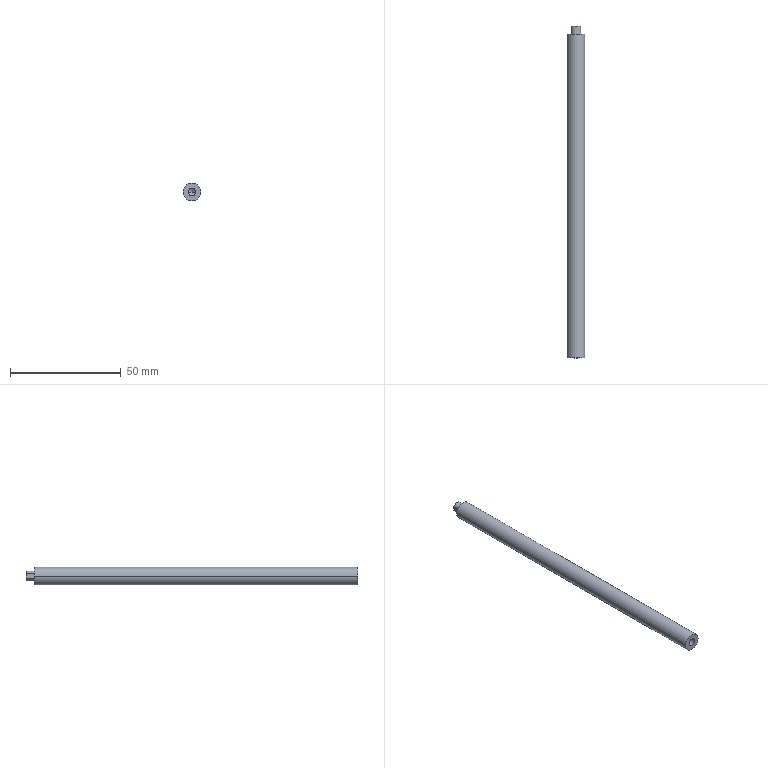Component | SolidWorks | 04LowerMaterialReceivingSwingAngleAssembly(3920)-1_04LowerMaterialReceivingDieAssembly(3920)-1_H2020022-0402-1-1 | 1 solid | 16 faces | box 8 x 150 x 8 mm | volume 7256 mm3 | cylinder 8 | cone 4 | plane 4 | commonest cylinder face diameters 3.3 x2 2.5 x2 4.5 x2 8 x2 | material 45#Steel
build123d program:
from build123d import *

# Parameters (mm, degrees)
SKETCH1_R             = 4
BOSS_EXTRUDE1_DEPTH   = 150
SKETCH2_OUTSIDE_W     = 40.086
SKETCH2_OUTSIDE_H     = 40.086
SKETCH2_OUTSIDE_R     = 2.25
CUT_EXTRUDE1_DEPTH    = 3.8
SKETCH3_W             = 6
SKETCH3_H             = 2
CUT_EXTRUDE2_DEPTH    = 3.8
M3_TAPPED_HOLE1_D     = 2.5
M3_TAPPED_HOLE1_DEPTH = 7.5
M3_TAPPED_HOLE1_TIP   = 0.7511
M4_TAPPED_HOLE1_D     = 3.3
M4_TAPPED_HOLE1_DEPTH = 13
M4_TAPPED_HOLE1_TIP   = 0.9914


with BuildPart() as part:
    # Sketch1 → Boss-Extrude1 (new body)
    with BuildSketch(Plane(origin=(0, 0, 0), x_dir=(1, 0, 0), z_dir=(0, 1, 0))):
        with Locations(Location((0, 0, 0), (0, 0, 270))):
            Circle(SKETCH1_R)
    extrude(amount=BOSS_EXTRUDE1_DEPTH)

    # Sketch2 outside → Cut-Extrude1 (cut)
    with BuildSketch(Plane(origin=(0, 150, 0), x_dir=(1, 0, 0), z_dir=(0, 1, 0))):
        Rectangle(SKETCH2_OUTSIDE_W, SKETCH2_OUTSIDE_H)
        with Locations(Location((0, 0, 0), (0, 0, 270))):
            Circle(SKETCH2_OUTSIDE_R, mode=Mode.SUBTRACT)
    extrude(amount=-CUT_EXTRUDE1_DEPTH, mode=Mode.SUBTRACT)

    # Sketch3 → Cut-Extrude2 (cut)
    with BuildSketch(Plane(origin=(0, 150, 0), x_dir=(1, 0, 0), z_dir=(0, 1, 0))):
        with Locations((0, 3)):
            Rectangle(SKETCH3_W, SKETCH3_H)
    extrude(amount=-CUT_EXTRUDE2_DEPTH, mode=Mode.SUBTRACT)

    # M3 Tapped Hole1
    with Locations(Plane(origin=(0, 150, 0), x_dir=(1, 0, 0), z_dir=(0, 1, 0))):
        with Locations((0, 0)):
            Hole(M3_TAPPED_HOLE1_D / 2, depth=M3_TAPPED_HOLE1_DEPTH)
            with Locations((0, 0, -(M3_TAPPED_HOLE1_DEPTH + M3_TAPPED_HOLE1_TIP / 2))):  # 118° drill point
                Cone(0, M3_TAPPED_HOLE1_D / 2, M3_TAPPED_HOLE1_TIP, mode=Mode.SUBTRACT)

    # M4 Tapped Hole1
    with Locations(Plane(origin=(0, 0, 0), x_dir=(-1, 0, 0), z_dir=(0, -1, 0))):
        with Locations((0, 0)):
            Hole(M4_TAPPED_HOLE1_D / 2, depth=M4_TAPPED_HOLE1_DEPTH)
            with Locations((0, 0, -(M4_TAPPED_HOLE1_DEPTH + M4_TAPPED_HOLE1_TIP / 2))):  # 118° drill point
                Cone(0, M4_TAPPED_HOLE1_D / 2, M4_TAPPED_HOLE1_TIP, mode=Mode.SUBTRACT)


solid = part.part

# Placed as in the assembly
solid = solid.moved(Location((0.03579, 124.813, 280.197), (0, 90, 0)))
STEP:
#1=COLOUR_RGB('',0.7922,0.8196,0.9333);
#2=FILL_AREA_STYLE_COLOUR('',#1);
#3=FILL_AREA_STYLE('',(#2));
#4=SURFACE_STYLE_FILL_AREA(#3);
#5=SURFACE_SIDE_STYLE('',(#4));
#6=SURFACE_STYLE_USAGE(.BOTH.,#5);
#7=PRESENTATION_STYLE_ASSIGNMENT((#6));
#8=CARTESIAN_POINT('',(0.06637,5.426,11.031));
#9=VERTEX_POINT('',#8);
#10=CARTESIAN_POINT('',(-0.06355,5.426,11.031));
#11=VERTEX_POINT('',#10);
#12=CARTESIAN_POINT('',(0.001409,5.426,11.031));
#13=DIRECTION('',(0.,-1.,0.));
#14=DIRECTION('',(-1.,0.,0.));
#15=AXIS2_PLACEMENT_3D('',#12,#13,#14);
#16=CIRCLE('',#15,0.06496);
#17=EDGE_CURVE('',#9,#11,#16,.T.);
#18=ORIENTED_EDGE('',*,*,#17,.F.);
#19=CARTESIAN_POINT('',(0.06637,4.914,11.031));
#20=VERTEX_POINT('',#19);
#21=CARTESIAN_POINT('',(0.06637,4.914,11.031));
#22=DIRECTION('',(0.,-1.,0.));
#23=VECTOR('',#22,39.37);
#24=LINE('',#21,#23);
#25=EDGE_CURVE('',#9,#20,#24,.T.);
#26=ORIENTED_EDGE('',*,*,#25,.T.);
#27=CARTESIAN_POINT('',(-0.06355,4.914,11.031));
#28=VERTEX_POINT('',#27);
#29=CARTESIAN_POINT('',(0.001409,4.914,11.031));
#30=DIRECTION('',(0.,-1.,0.));
#31=DIRECTION('',(-1.,0.,0.));
#32=AXIS2_PLACEMENT_3D('',#29,#30,#31);
#33=CIRCLE('',#32,0.06496);
#34=EDGE_CURVE('',#20,#28,#33,.T.);
#35=ORIENTED_EDGE('',*,*,#34,.T.);
#36=CARTESIAN_POINT('',(-0.06355,4.914,11.031));
#37=DIRECTION('',(0.,-1.,0.));
#38=VECTOR('',#37,39.37);
#39=LINE('',#36,#38);
#40=EDGE_CURVE('',#11,#28,#39,.T.);
#41=ORIENTED_EDGE('',*,*,#40,.F.);
#42=EDGE_LOOP('',(#18,#26,#35,#41));
#43=FACE_OUTER_BOUND('',#42,.T.);
#44=CARTESIAN_POINT('',(0.001409,4.914,11.031));
#45=DIRECTION('',(0.,-1.,0.));
#46=DIRECTION('',(-1.,0.,0.));
#47=AXIS2_PLACEMENT_3D('',#44,#45,#46);
#48=CYLINDRICAL_SURFACE('',#47,0.06496);
#49=ADVANCED_FACE('',(#43),#48,.F.);
#50=CARTESIAN_POINT('',(0.001409,5.465,11.031));
#51=VERTEX_POINT('',#50);
#52=CARTESIAN_POINT('',(-0.06355,5.426,11.031));
#53=DIRECTION('',(-0.8572,-0.515,0.));
#54=VECTOR('',#53,39.37);
#55=LINE('',#52,#54);
#56=EDGE_CURVE('',#51,#11,#55,.T.);
#57=ORIENTED_EDGE('',*,*,#56,.F.);
#58=CARTESIAN_POINT('',(0.06637,5.426,11.031));
#59=DIRECTION('',(0.8572,-0.515,-0.));
#60=VECTOR('',#59,39.37);
#61=LINE('',#58,#60);
#62=EDGE_CURVE('',#51,#9,#61,.T.);
#63=ORIENTED_EDGE('',*,*,#62,.T.);
#64=ORIENTED_EDGE('',*,*,#17,.T.);
#65=EDGE_LOOP('',(#57,#63,#64));
#66=FACE_OUTER_BOUND('',#65,.T.);
#67=CARTESIAN_POINT('',(0.001409,5.426,11.031));
#68=DIRECTION('',(0.,-1.,0.));
#69=DIRECTION('',(-1.,0.,0.));
#70=AXIS2_PLACEMENT_3D('',#67,#68,#69);
#71=CONICAL_SURFACE('',#70,0.06496,1.03);
#72=ADVANCED_FACE('',(#66),#71,.F.);
#73=CARTESIAN_POINT('',(-0.0478,10.524,11.031));
#74=VERTEX_POINT('',#73);
#75=CARTESIAN_POINT('',(0.05062,10.524,11.031));
#76=VERTEX_POINT('',#75);
#77=CARTESIAN_POINT('',(0.001409,10.524,11.031));
#78=DIRECTION('',(0.,1.,0.));
#79=DIRECTION('',(1.,0.,0.));
#80=AXIS2_PLACEMENT_3D('',#77,#78,#79);
#81=CIRCLE('',#80,0.04921);
#82=EDGE_CURVE('',#74,#76,#81,.T.);
#83=ORIENTED_EDGE('',*,*,#82,.F.);
#84=CARTESIAN_POINT('',(-0.0478,10.819,11.031));
#85=VERTEX_POINT('',#84);
#86=CARTESIAN_POINT('',(-0.0478,10.819,11.031));
#87=DIRECTION('',(0.,1.,0.));
#88=VECTOR('',#87,39.37);
#89=LINE('',#86,#88);
#90=EDGE_CURVE('',#74,#85,#89,.T.);
#91=ORIENTED_EDGE('',*,*,#90,.T.);
#92=CARTESIAN_POINT('',(0.05062,10.819,11.031));
#93=VERTEX_POINT('',#92);
#94=CARTESIAN_POINT('',(0.001409,10.819,11.031));
#95=DIRECTION('',(0.,1.,0.));
#96=DIRECTION('',(1.,0.,0.));
#97=AXIS2_PLACEMENT_3D('',#94,#95,#96);
#98=CIRCLE('',#97,0.04921);
#99=EDGE_CURVE('',#85,#93,#98,.T.);
#100=ORIENTED_EDGE('',*,*,#99,.T.);
#101=CARTESIAN_POINT('',(0.05062,10.819,11.031));
#102=DIRECTION('',(0.,1.,0.));
#103=VECTOR('',#102,39.37);
#104=LINE('',#101,#103);
#105=EDGE_CURVE('',#76,#93,#104,.T.);
#106=ORIENTED_EDGE('',*,*,#105,.F.);
#107=EDGE_LOOP('',(#83,#91,#100,#106));
#108=FACE_OUTER_BOUND('',#107,.T.);
#109=CARTESIAN_POINT('',(0.001409,10.819,11.031));
#110=DIRECTION('',(0.,1.,0.));
#111=DIRECTION('',(1.,0.,0.));
#112=AXIS2_PLACEMENT_3D('',#109,#110,#111);
#113=CYLINDRICAL_SURFACE('',#112,0.04921);
#114=ADVANCED_FACE('',(#108),#113,.F.);
#115=CARTESIAN_POINT('',(0.001409,10.495,11.031));
#116=VERTEX_POINT('',#115);
#117=CARTESIAN_POINT('',(0.05062,10.524,11.031));
#118=DIRECTION('',(0.8572,0.515,-0.));
#119=VECTOR('',#118,39.37);
#120=LINE('',#117,#119);
#121=EDGE_CURVE('',#116,#76,#120,.T.);
#122=ORIENTED_EDGE('',*,*,#121,.F.);
#123=CARTESIAN_POINT('',(-0.0478,10.524,11.031));
#124=DIRECTION('',(-0.8572,0.515,0.));
#125=VECTOR('',#124,39.37);
#126=LINE('',#123,#125);
#127=EDGE_CURVE('',#116,#74,#126,.T.);
#128=ORIENTED_EDGE('',*,*,#127,.T.);
#129=ORIENTED_EDGE('',*,*,#82,.T.);
#130=EDGE_LOOP('',(#122,#128,#129));
#131=FACE_OUTER_BOUND('',#130,.T.);
#132=CARTESIAN_POINT('',(0.001409,10.524,11.031));
#133=DIRECTION('',(0.,1.,0.));
#134=DIRECTION('',(1.,0.,0.));
#135=AXIS2_PLACEMENT_3D('',#132,#133,#134);
#136=CONICAL_SURFACE('',#135,0.04921,1.03);
#137=ADVANCED_FACE('',(#131),#136,.F.);
#138=CARTESIAN_POINT('',(-0.07733,10.67,11.072));
#139=VERTEX_POINT('',#138);
#140=CARTESIAN_POINT('',(0.08999,10.67,11.031));
#141=VERTEX_POINT('',#140);
#142=CARTESIAN_POINT('',(0.001409,10.67,11.031));
#143=DIRECTION('',(0.,1.,0.));
#144=DIRECTION('',(1.,0.,0.));
#145=AXIS2_PLACEMENT_3D('',#142,#143,#144);
#146=CIRCLE('',#145,0.08858);
#147=EDGE_CURVE('',#139,#141,#146,.T.);
#148=ORIENTED_EDGE('',*,*,#147,.T.);
#149=CARTESIAN_POINT('',(0.08999,10.819,11.031));
#150=VERTEX_POINT('',#149);
#151=CARTESIAN_POINT('',(0.08999,10.67,11.031));
#152=DIRECTION('',(0.,1.,0.));
#153=VECTOR('',#152,39.37);
#154=LINE('',#151,#153);
#155=EDGE_CURVE('',#141,#150,#154,.T.);
#156=ORIENTED_EDGE('',*,*,#155,.T.);
#157=CARTESIAN_POINT('',(-0.07733,10.819,11.072));
#158=VERTEX_POINT('',#157);
#159=CARTESIAN_POINT('',(0.001409,10.819,11.031));
#160=DIRECTION('',(0.,1.,0.));
#161=DIRECTION('',(1.,0.,0.));
#162=AXIS2_PLACEMENT_3D('',#159,#160,#161);
#163=CIRCLE('',#162,0.08858);
#164=EDGE_CURVE('',#158,#150,#163,.T.);
#165=ORIENTED_EDGE('',*,*,#164,.F.);
#166=CARTESIAN_POINT('',(-0.07733,10.67,11.072));
#167=DIRECTION('',(0.,1.,0.));
#168=VECTOR('',#167,39.37);
#169=LINE('',#166,#168);
#170=EDGE_CURVE('',#139,#158,#169,.T.);
#171=ORIENTED_EDGE('',*,*,#170,.F.);
#172=EDGE_LOOP('',(#148,#156,#165,#171));
#173=FACE_OUTER_BOUND('',#172,.T.);
#174=CARTESIAN_POINT('',(0.001409,10.67,11.031));
#175=DIRECTION('',(0.,1.,0.));
#176=DIRECTION('',(1.,0.,0.));
#177=AXIS2_PLACEMENT_3D('',#174,#175,#176);
#178=CYLINDRICAL_SURFACE('',#177,0.08858);
#179=ADVANCED_FACE('',(#173),#178,.T.);
#180=CARTESIAN_POINT('',(0.1589,10.67,11.031));
#181=VERTEX_POINT('',#180);
#182=CARTESIAN_POINT('',(-0.1561,10.67,11.031));
#183=VERTEX_POINT('',#182);
#184=CARTESIAN_POINT('',(0.001409,10.67,11.031));
#185=DIRECTION('',(0.,1.,0.));
#186=DIRECTION('',(1.,0.,0.));
#187=AXIS2_PLACEMENT_3D('',#184,#185,#186);
#188=CIRCLE('',#187,0.1575);
#189=EDGE_CURVE('',#181,#183,#188,.T.);
#190=ORIENTED_EDGE('',*,*,#189,.F.);
#191=CARTESIAN_POINT('',(0.1589,4.914,11.031));
#192=VERTEX_POINT('',#191);
#193=CARTESIAN_POINT('',(0.1589,10.819,11.031));
#194=DIRECTION('',(0.,-1.,0.));
#195=VECTOR('',#194,39.37);
#196=LINE('',#193,#195);
#197=EDGE_CURVE('',#181,#192,#196,.T.);
#198=ORIENTED_EDGE('',*,*,#197,.T.);
#199=CARTESIAN_POINT('',(-0.1561,4.914,11.031));
#200=VERTEX_POINT('',#199);
#201=CARTESIAN_POINT('',(0.001409,4.914,11.031));
#202=DIRECTION('',(0.,1.,0.));
#203=DIRECTION('',(1.,0.,0.));
#204=AXIS2_PLACEMENT_3D('',#201,#202,#203);
#205=CIRCLE('',#204,0.1575);
#206=EDGE_CURVE('',#192,#200,#205,.T.);
#207=ORIENTED_EDGE('',*,*,#206,.T.);
#208=CARTESIAN_POINT('',(-0.1561,10.819,11.031));
#209=DIRECTION('',(0.,-1.,0.));
#210=VECTOR('',#209,39.37);
#211=LINE('',#208,#210);
#212=EDGE_CURVE('',#183,#200,#211,.T.);
#213=ORIENTED_EDGE('',*,*,#212,.F.);
#214=EDGE_LOOP('',(#190,#198,#207,#213));
#215=FACE_OUTER_BOUND('',#214,.T.);
#216=CARTESIAN_POINT('',(0.001409,10.819,11.031));
#217=DIRECTION('',(0.,-1.,0.));
#218=DIRECTION('',(-1.,0.,0.));
#219=AXIS2_PLACEMENT_3D('',#216,#217,#218);
#220=CYLINDRICAL_SURFACE('',#219,0.1575);
#221=ADVANCED_FACE('',(#215),#220,.T.);
#222=ORIENTED_EDGE('',*,*,#197,.F.);
#223=CARTESIAN_POINT('',(0.001409,10.67,11.031));
#224=DIRECTION('',(0.,1.,0.));
#225=DIRECTION('',(1.,0.,0.));
#226=AXIS2_PLACEMENT_3D('',#223,#224,#225);
#227=CIRCLE('',#226,0.1575);
#228=EDGE_CURVE('',#183,#181,#227,.T.);
#229=ORIENTED_EDGE('',*,*,#228,.F.);
#230=ORIENTED_EDGE('',*,*,#212,.T.);
#231=CARTESIAN_POINT('',(0.001409,4.914,11.031));
#232=DIRECTION('',(0.,1.,0.));
#233=DIRECTION('',(1.,0.,0.));
#234=AXIS2_PLACEMENT_3D('',#231,#232,#233);
#235=CIRCLE('',#234,0.1575);
#236=EDGE_CURVE('',#200,#192,#235,.T.);
#237=ORIENTED_EDGE('',*,*,#236,.T.);
#238=EDGE_LOOP('',(#222,#229,#230,#237));
#239=FACE_OUTER_BOUND('',#238,.T.);
#240=CARTESIAN_POINT('',(0.001409,10.819,11.031));
#241=DIRECTION('',(0.,-1.,0.));
#242=DIRECTION('',(-1.,0.,0.));
#243=AXIS2_PLACEMENT_3D('',#240,#241,#242);
#244=CYLINDRICAL_SURFACE('',#243,0.1575);
#245=ADVANCED_FACE('',(#239),#244,.T.);
#246=CARTESIAN_POINT('',(0.001409,4.914,11.031));
#247=DIRECTION('',(0.,-1.,0.));
#248=DIRECTION('',(-1.,0.,0.));
#249=AXIS2_PLACEMENT_3D('',#246,#247,#248);
#250=CIRCLE('',#249,0.06496);
#251=EDGE_CURVE('',#28,#20,#250,.T.);
#252=ORIENTED_EDGE('',*,*,#251,.F.);
#253=ORIENTED_EDGE('',*,*,#34,.F.);
#254=EDGE_LOOP('',(#252,#253));
#255=FACE_BOUND('',#254,.T.);
#256=ORIENTED_EDGE('',*,*,#236,.F.);
#257=ORIENTED_EDGE('',*,*,#206,.F.);
#258=EDGE_LOOP('',(#256,#257));
#259=FACE_OUTER_BOUND('',#258,.T.);
#260=CARTESIAN_POINT('',(0.001409,4.914,11.031));
#261=DIRECTION('',(0.,1.,0.));
#262=DIRECTION('',(1.,0.,-0.));
#263=AXIS2_PLACEMENT_3D('',#260,#261,#262);
#264=PLANE('',#263);
#265=ADVANCED_FACE('',(#255,#259),#264,.F.);
#266=ORIENTED_EDGE('',*,*,#228,.T.);
#267=ORIENTED_EDGE('',*,*,#189,.T.);
#268=EDGE_LOOP('',(#266,#267));
#269=FACE_OUTER_BOUND('',#268,.T.);
#270=ORIENTED_EDGE('',*,*,#147,.F.);
#271=CARTESIAN_POINT('',(-0.07733,10.67,10.991));
#272=VERTEX_POINT('',#271);
#273=CARTESIAN_POINT('',(-0.07733,10.67,11.149));
#274=DIRECTION('',(0.,0.,1.));
#275=VECTOR('',#274,39.37);
#276=LINE('',#273,#275);
#277=EDGE_CURVE('',#272,#139,#276,.T.);
#278=ORIENTED_EDGE('',*,*,#277,.F.);
#279=CARTESIAN_POINT('',(0.001409,10.67,11.031));
#280=DIRECTION('',(0.,1.,0.));
#281=DIRECTION('',(1.,0.,0.));
#282=AXIS2_PLACEMENT_3D('',#279,#280,#281);
#283=CIRCLE('',#282,0.08858);
#284=EDGE_CURVE('',#141,#272,#283,.T.);
#285=ORIENTED_EDGE('',*,*,#284,.F.);
#286=EDGE_LOOP('',(#270,#278,#285));
#287=FACE_BOUND('',#286,.T.);
#288=CARTESIAN_POINT('',(0.001409,10.67,11.031));
#289=DIRECTION('',(0.,1.,0.));
#290=DIRECTION('',(1.,0.,-0.));
#291=AXIS2_PLACEMENT_3D('',#288,#289,#290);
#292=PLANE('',#291);
#293=ADVANCED_FACE('',(#269,#287),#292,.T.);
#294=ORIENTED_EDGE('',*,*,#155,.F.);
#295=ORIENTED_EDGE('',*,*,#284,.T.);
#296=CARTESIAN_POINT('',(-0.07733,10.819,10.991));
#297=VERTEX_POINT('',#296);
#298=CARTESIAN_POINT('',(-0.07733,10.67,10.991));
#299=DIRECTION('',(0.,-1.,0.));
#300=VECTOR('',#299,39.37);
#301=LINE('',#298,#300);
#302=EDGE_CURVE('',#297,#272,#301,.T.);
#303=ORIENTED_EDGE('',*,*,#302,.F.);
#304=CARTESIAN_POINT('',(0.001409,10.819,11.031));
#305=DIRECTION('',(0.,1.,0.));
#306=DIRECTION('',(1.,0.,0.));
#307=AXIS2_PLACEMENT_3D('',#304,#305,#306);
#308=CIRCLE('',#307,0.08858);
#309=EDGE_CURVE('',#150,#297,#308,.T.);
#310=ORIENTED_EDGE('',*,*,#309,.F.);
#311=EDGE_LOOP('',(#294,#295,#303,#310));
#312=FACE_OUTER_BOUND('',#311,.T.);
#313=CARTESIAN_POINT('',(0.001409,10.67,11.031));
#314=DIRECTION('',(0.,1.,0.));
#315=DIRECTION('',(1.,0.,0.));
#316=AXIS2_PLACEMENT_3D('',#313,#314,#315);
#317=CYLINDRICAL_SURFACE('',#316,0.08858);
#318=ADVANCED_FACE('',(#312),#317,.T.);
#319=CARTESIAN_POINT('',(0.001409,10.819,11.031));
#320=DIRECTION('',(0.,1.,0.));
#321=DIRECTION('',(1.,0.,0.));
#322=AXIS2_PLACEMENT_3D('',#319,#320,#321);
#323=CIRCLE('',#322,0.04921);
#324=EDGE_CURVE('',#93,#85,#323,.T.);
#325=ORIENTED_EDGE('',*,*,#324,.F.);
#326=ORIENTED_EDGE('',*,*,#99,.F.);
#327=EDGE_LOOP('',(#325,#326));
#328=FACE_BOUND('',#327,.T.);
#329=CARTESIAN_POINT('',(-0.07733,10.819,11.031));
#330=DIRECTION('',(-0.,0.,-1.));
#331=VECTOR('',#330,39.37);
#332=LINE('',#329,#331);
#333=EDGE_CURVE('',#158,#297,#332,.T.);
#334=ORIENTED_EDGE('',*,*,#333,.F.);
#335=ORIENTED_EDGE('',*,*,#164,.T.);
#336=ORIENTED_EDGE('',*,*,#309,.T.);
#337=EDGE_LOOP('',(#334,#335,#336));
#338=FACE_OUTER_BOUND('',#337,.T.);
#339=CARTESIAN_POINT('',(0.001409,10.819,11.031));
#340=DIRECTION('',(0.,1.,0.));
#341=DIRECTION('',(1.,0.,-0.));
#342=AXIS2_PLACEMENT_3D('',#339,#340,#341);
#343=PLANE('',#342);
#344=ADVANCED_FACE('',(#328,#338),#343,.T.);
#345=ORIENTED_EDGE('',*,*,#302,.T.);
#346=ORIENTED_EDGE('',*,*,#277,.T.);
#347=ORIENTED_EDGE('',*,*,#170,.T.);
#348=ORIENTED_EDGE('',*,*,#333,.T.);
#349=EDGE_LOOP('',(#345,#346,#347,#348));
#350=FACE_OUTER_BOUND('',#349,.T.);
#351=CARTESIAN_POINT('',(-0.07733,10.421,11.149));
#352=DIRECTION('',(1.,0.,-0.));
#353=DIRECTION('',(-0.,0.,-1.));
#354=AXIS2_PLACEMENT_3D('',#351,#352,#353);
#355=PLANE('',#354);
#356=ADVANCED_FACE('',(#350),#355,.F.);
#357=ORIENTED_EDGE('',*,*,#127,.F.);
#358=ORIENTED_EDGE('',*,*,#121,.T.);
#359=CARTESIAN_POINT('',(0.001409,10.524,11.031));
#360=DIRECTION('',(0.,1.,0.));
#361=DIRECTION('',(1.,0.,0.));
#362=AXIS2_PLACEMENT_3D('',#359,#360,#361);
#363=CIRCLE('',#362,0.04921);
#364=EDGE_CURVE('',#76,#74,#363,.T.);
#365=ORIENTED_EDGE('',*,*,#364,.T.);
#366=EDGE_LOOP('',(#357,#358,#365));
#367=FACE_OUTER_BOUND('',#366,.T.);
#368=CARTESIAN_POINT('',(0.001409,10.524,11.031));
#369=DIRECTION('',(0.,1.,0.));
#370=DIRECTION('',(1.,0.,0.));
#371=AXIS2_PLACEMENT_3D('',#368,#369,#370);
#372=CONICAL_SURFACE('',#371,0.04921,1.03);
#373=ADVANCED_FACE('',(#367),#372,.F.);
#374=ORIENTED_EDGE('',*,*,#90,.F.);
#375=ORIENTED_EDGE('',*,*,#364,.F.);
#376=ORIENTED_EDGE('',*,*,#105,.T.);
#377=ORIENTED_EDGE('',*,*,#324,.T.);
#378=EDGE_LOOP('',(#374,#375,#376,#377));
#379=FACE_OUTER_BOUND('',#378,.T.);
#380=CARTESIAN_POINT('',(0.001409,10.819,11.031));
#381=DIRECTION('',(0.,1.,0.));
#382=DIRECTION('',(1.,0.,0.));
#383=AXIS2_PLACEMENT_3D('',#380,#381,#382);
#384=CYLINDRICAL_SURFACE('',#383,0.04921);
#385=ADVANCED_FACE('',(#379),#384,.F.);
#386=ORIENTED_EDGE('',*,*,#62,.F.);
#387=ORIENTED_EDGE('',*,*,#56,.T.);
#388=CARTESIAN_POINT('',(0.001409,5.426,11.031));
#389=DIRECTION('',(0.,-1.,0.));
#390=DIRECTION('',(-1.,0.,0.));
#391=AXIS2_PLACEMENT_3D('',#388,#389,#390);
#392=CIRCLE('',#391,0.06496);
#393=EDGE_CURVE('',#11,#9,#392,.T.);
#394=ORIENTED_EDGE('',*,*,#393,.T.);
#395=EDGE_LOOP('',(#386,#387,#394));
#396=FACE_OUTER_BOUND('',#395,.T.);
#397=CARTESIAN_POINT('',(0.001409,5.426,11.031));
#398=DIRECTION('',(0.,-1.,0.));
#399=DIRECTION('',(-1.,0.,0.));
#400=AXIS2_PLACEMENT_3D('',#397,#398,#399);
#401=CONICAL_SURFACE('',#400,0.06496,1.03);
#402=ADVANCED_FACE('',(#396),#401,.F.);
#403=ORIENTED_EDGE('',*,*,#25,.F.);
#404=ORIENTED_EDGE('',*,*,#393,.F.);
#405=ORIENTED_EDGE('',*,*,#40,.T.);
#406=ORIENTED_EDGE('',*,*,#251,.T.);
#407=EDGE_LOOP('',(#403,#404,#405,#406));
#408=FACE_OUTER_BOUND('',#407,.T.);
#409=CARTESIAN_POINT('',(0.001409,4.914,11.031));
#410=DIRECTION('',(0.,-1.,0.));
#411=DIRECTION('',(-1.,0.,0.));
#412=AXIS2_PLACEMENT_3D('',#409,#410,#411);
#413=CYLINDRICAL_SURFACE('',#412,0.06496);
#414=ADVANCED_FACE('',(#408),#413,.F.);
#415=CLOSED_SHELL('',(#49,#72,#114,#137,#179,#221,#245,#265,#293,#318,#344,#356,#373,#385,#402,#414));
#416=MANIFOLD_SOLID_BREP('',#415);
#417=STYLED_ITEM('',(#7),#416);
#418=PRESENTATION_LAYER_ASSIGNMENT('','',(#417));
#419=(LENGTH_UNIT()NAMED_UNIT(*)SI_UNIT($,.METRE.));
#420=LENGTH_MEASURE_WITH_UNIT(LENGTH_MEASURE(0.0254),#419);
#421=DIMENSIONAL_EXPONENTS(1.,0.,0.,0.,0.,0.,0.);
#422=(CONVERSION_BASED_UNIT('',#420)LENGTH_UNIT()NAMED_UNIT(#421));
#423=UNCERTAINTY_MEASURE_WITH_UNIT(LENGTH_MEASURE(0.00001),#422,'','');
#424=(NAMED_UNIT(*)PLANE_ANGLE_UNIT()SI_UNIT($,.RADIAN.));
#425=(NAMED_UNIT(*)SI_UNIT($,.STERADIAN.)SOLID_ANGLE_UNIT());
#426=(GEOMETRIC_REPRESENTATION_CONTEXT(3)GLOBAL_UNCERTAINTY_ASSIGNED_CONTEXT((#423))GLOBAL_UNIT_ASSIGNED_CONTEXT((#422,#424,#425))REPRESENTATION_CONTEXT('',''));
#427=MECHANICAL_DESIGN_GEOMETRIC_PRESENTATION_REPRESENTATION('',(#417),#426);
#428=CARTESIAN_POINT('',(0.,0.,0.));
#429=DIRECTION('',(0.,0.,1.));
#430=DIRECTION('',(1.,0.,0.));
#431=AXIS2_PLACEMENT_3D('',#428,#429,#430);
#432=(LENGTH_UNIT()NAMED_UNIT(*)SI_UNIT($,.METRE.));
#433=LENGTH_MEASURE_WITH_UNIT(LENGTH_MEASURE(0.0254),#432);
#434=DIMENSIONAL_EXPONENTS(1.,0.,0.,0.,0.,0.,0.);
#435=(CONVERSION_BASED_UNIT('',#433)LENGTH_UNIT()NAMED_UNIT(#434));
#436=UNCERTAINTY_MEASURE_WITH_UNIT(LENGTH_MEASURE(0.00001),#435,'','');
#437=(NAMED_UNIT(*)PLANE_ANGLE_UNIT()SI_UNIT($,.RADIAN.));
#438=(NAMED_UNIT(*)SI_UNIT($,.STERADIAN.)SOLID_ANGLE_UNIT());
#439=(GEOMETRIC_REPRESENTATION_CONTEXT(3)GLOBAL_UNCERTAINTY_ASSIGNED_CONTEXT((#436))GLOBAL_UNIT_ASSIGNED_CONTEXT((#435,#437,#438))REPRESENTATION_CONTEXT('',''));
#440=ADVANCED_BREP_SHAPE_REPRESENTATION('',(#416,#431),#439);